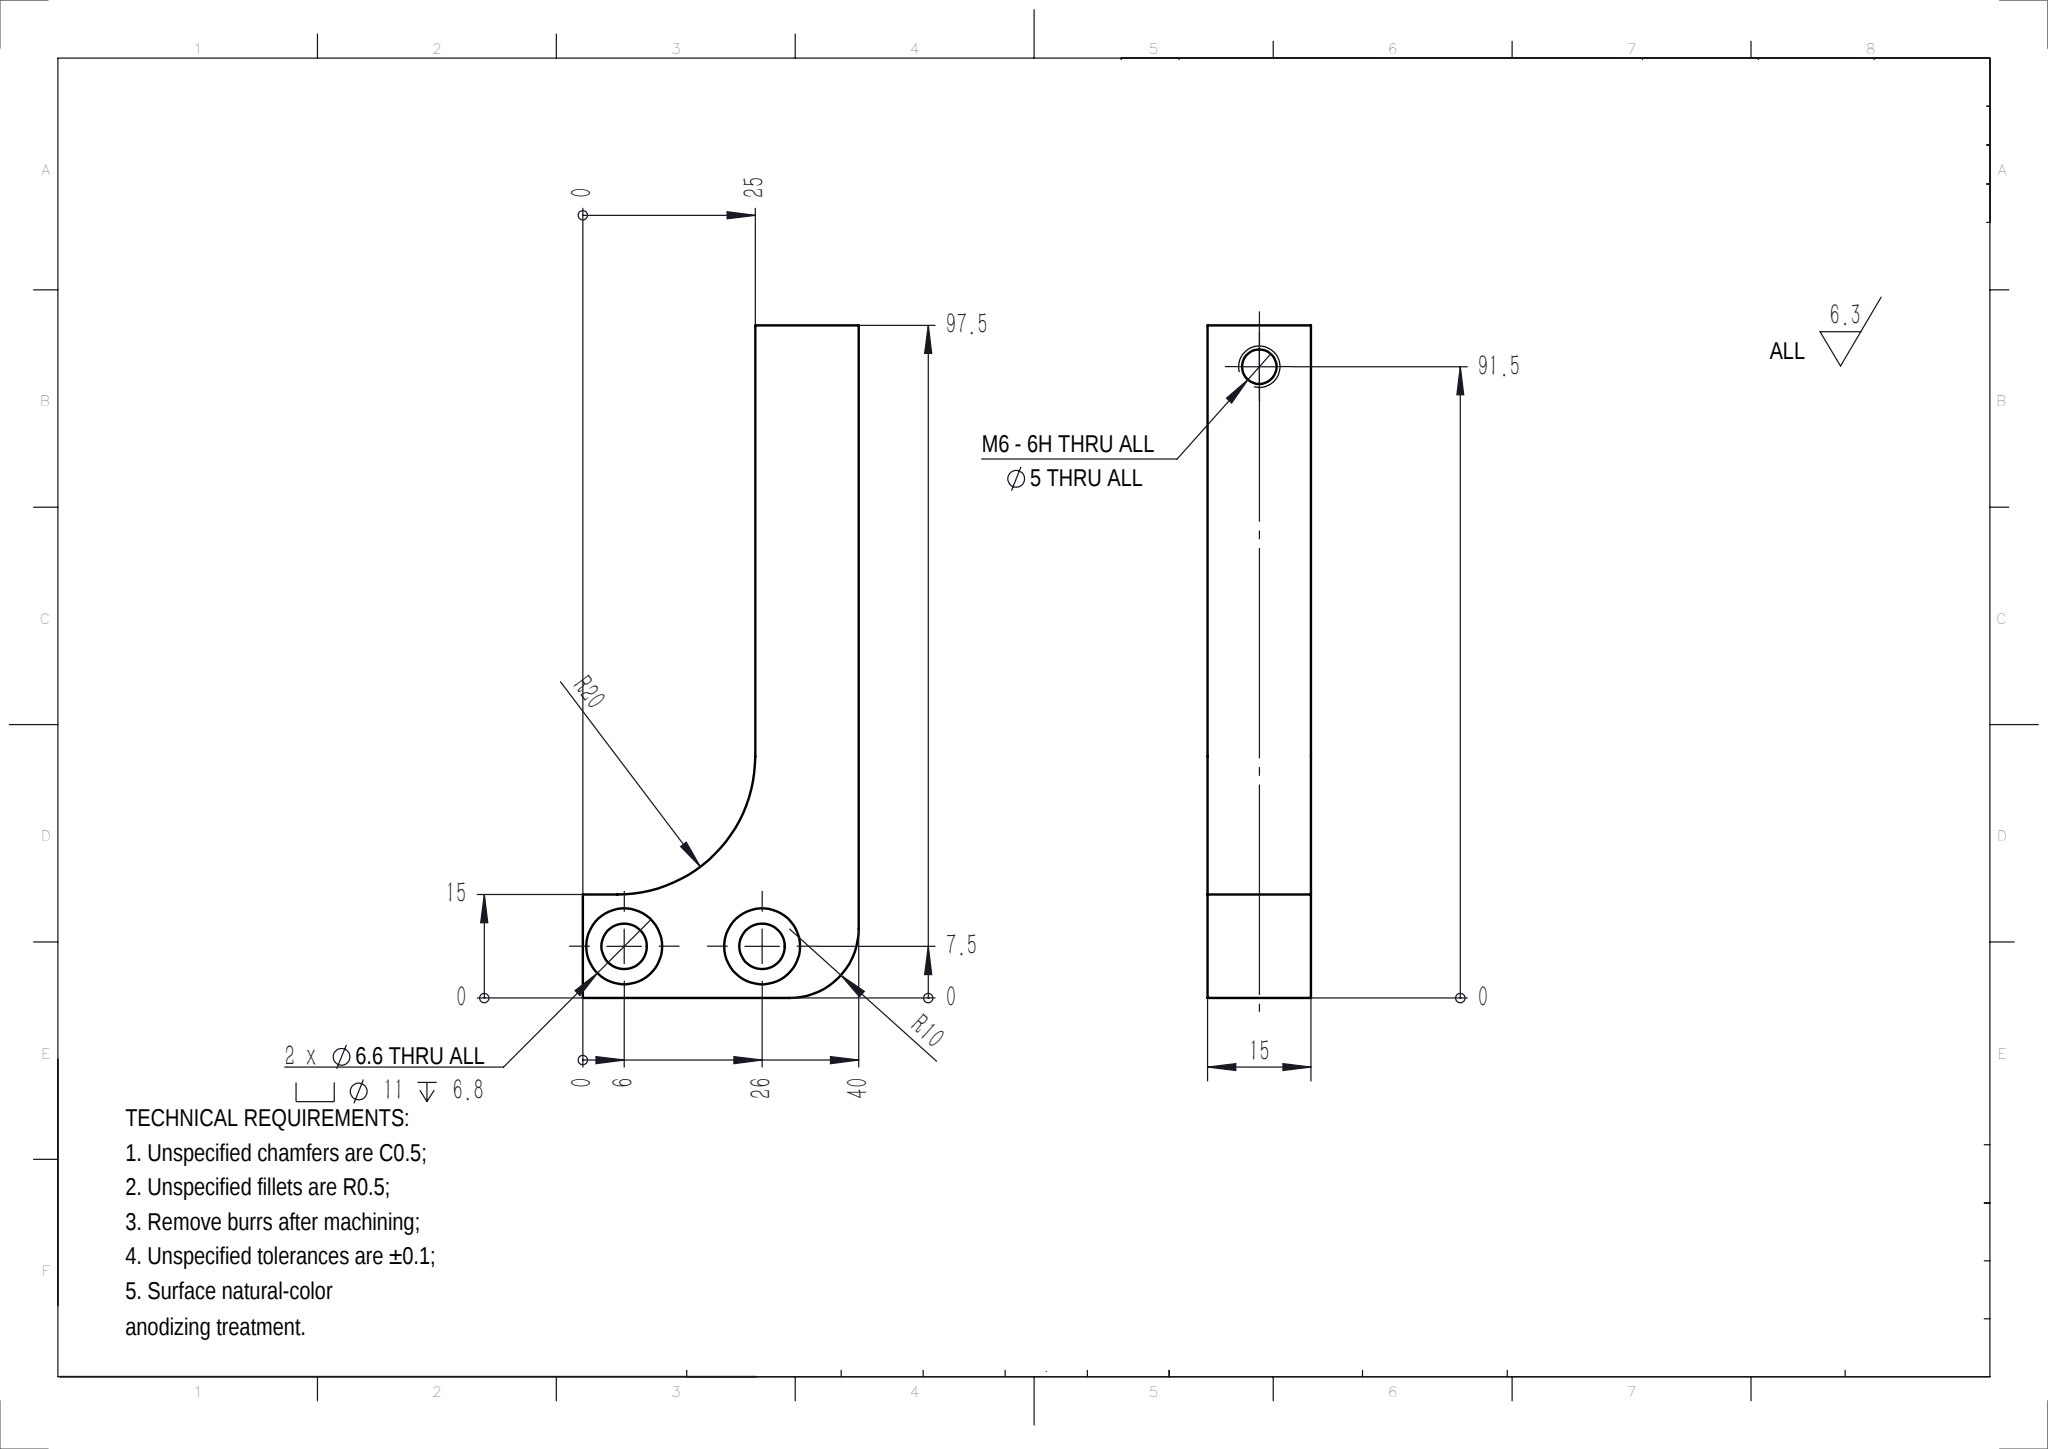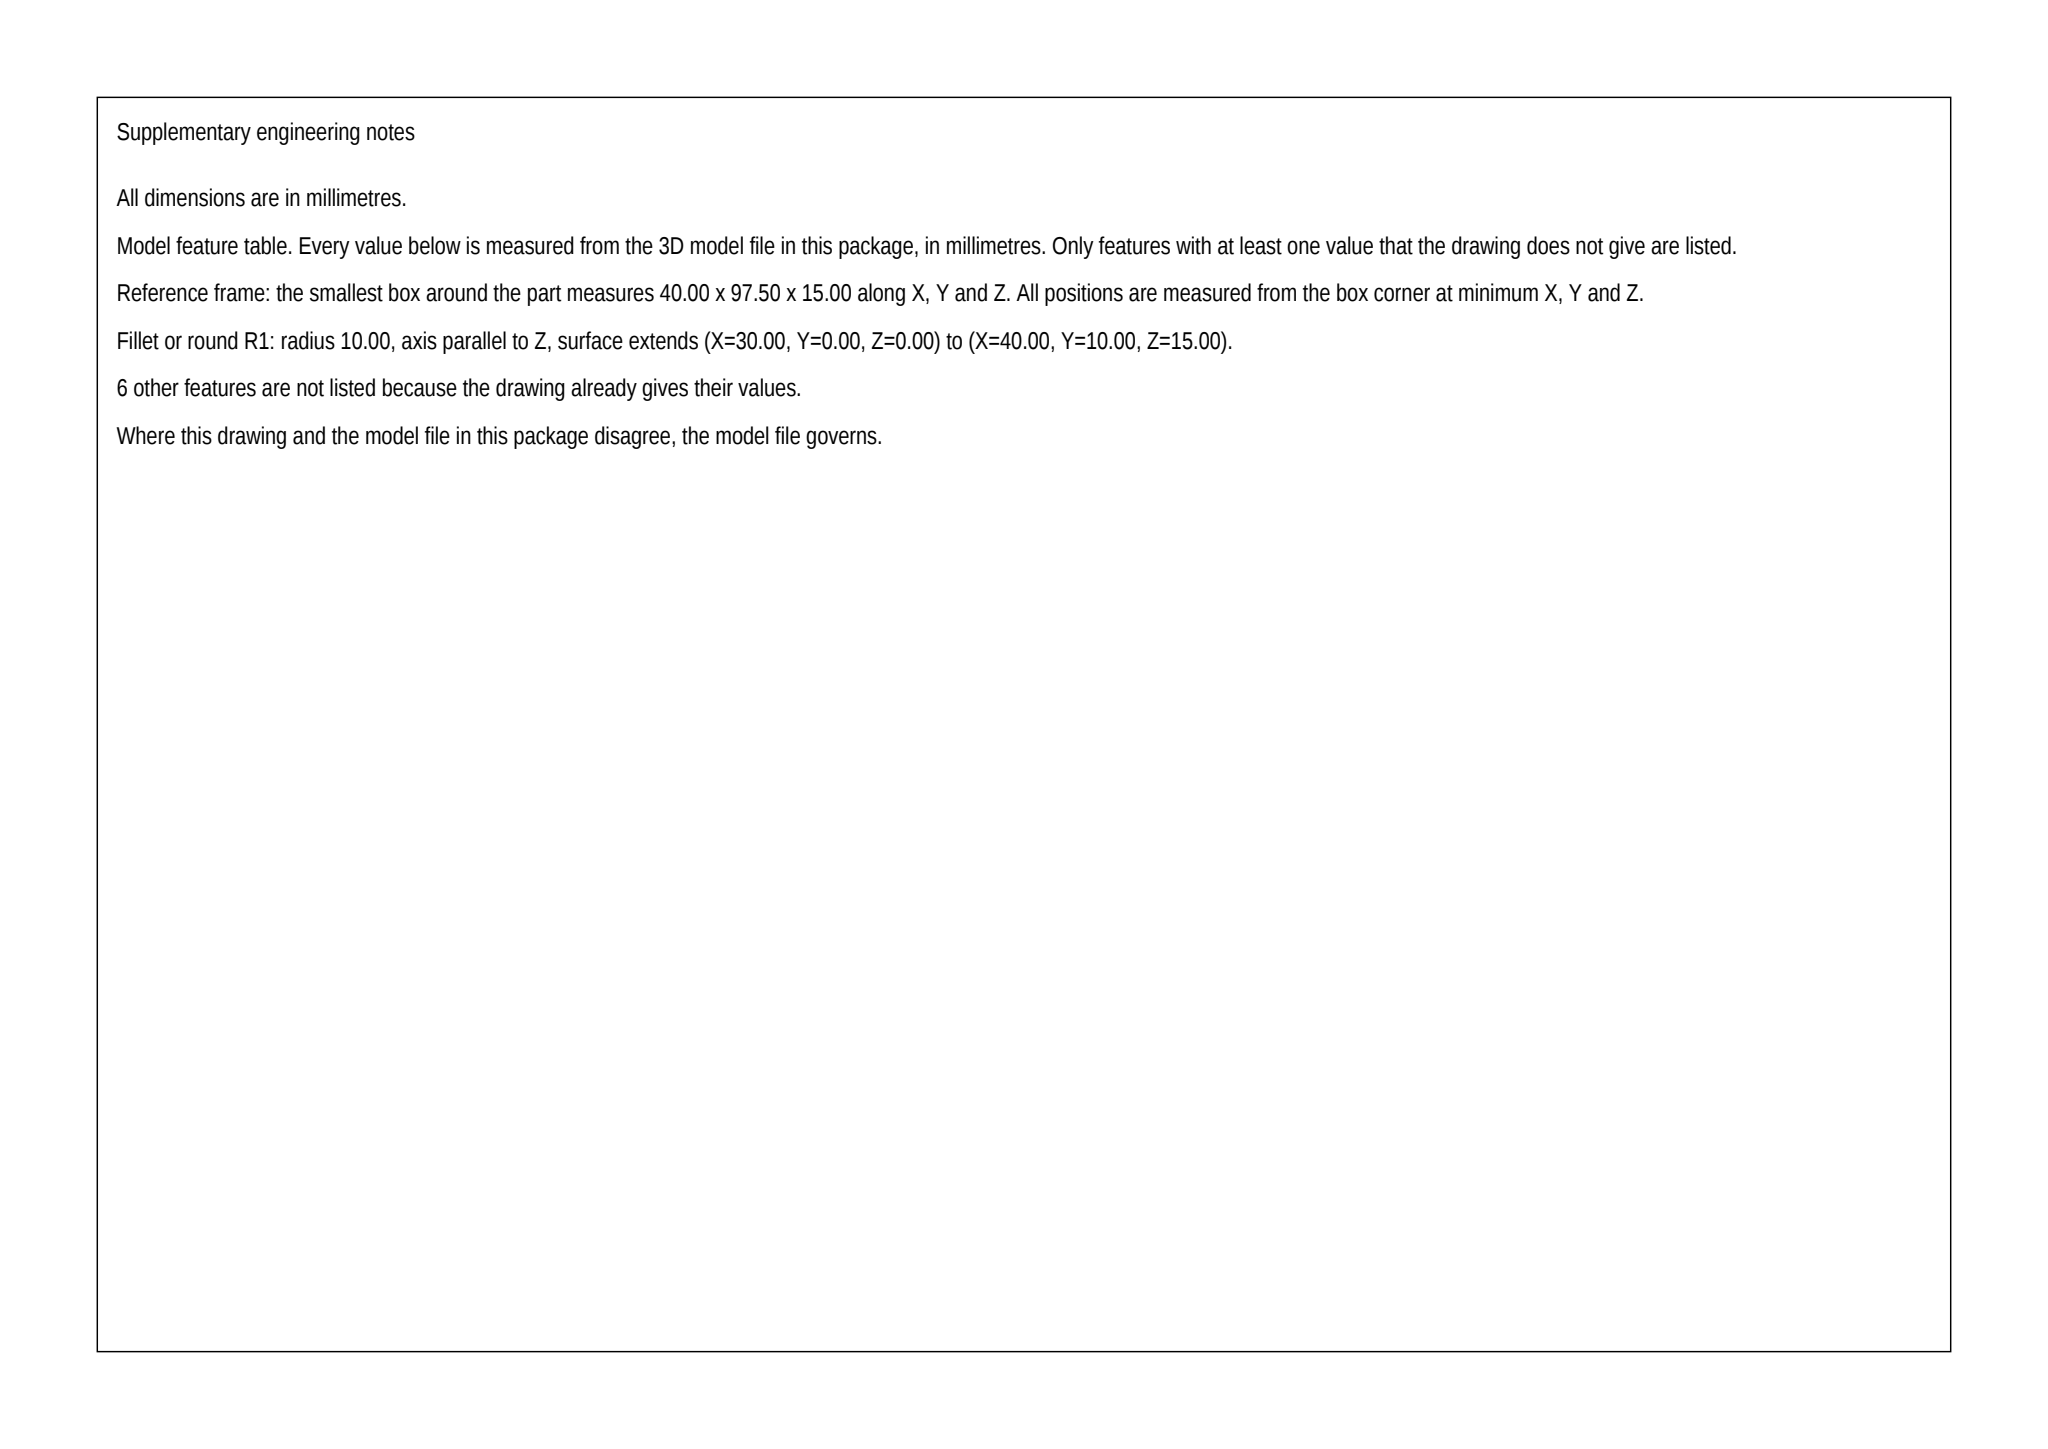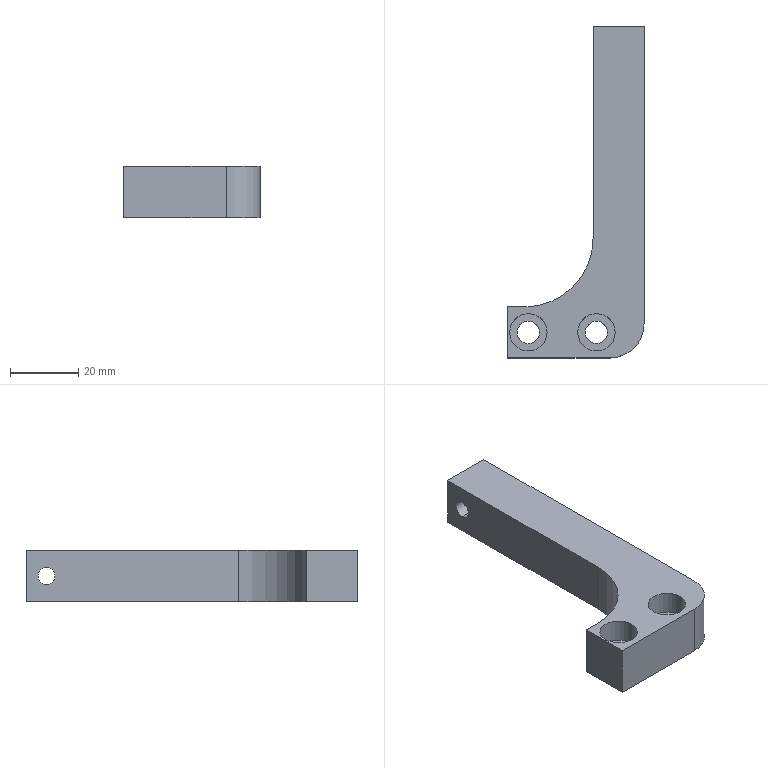Part | SolidWorks | mm | 1 solid | 22 faces | box 40 x 97.5 x 15 mm | volume 26380 mm3 | cylinder 12 | plane 10 | commonest cylinder face diameters 11 x4 6.6 x4 5 x2 40 x1 20 x1
build123d program:
from build123d import *

# Parameters (mm, degrees)
BOSS_EXTRUDE1_DEPTH                               = 7.5
HOLE_SIZE_ACCORDING_TO_HEXAGON_SOCKET_D           = 6.6
HOLE_SIZE_ACCORDING_TO_HEXAGON_SOCKET_CBORE_D     = 11
HOLE_SIZE_ACCORDING_TO_HEXAGON_SOCKET_CBORE_DEPTH = 6.8
M6_TAPPED_HOLE1_D                                 = 5
FILLET1_R                                         = 20
FILLET2_R                                         = 10


with BuildPart() as part:
    # Sketch1 → Boss-Extrude1 (new, symmetric)
    with BuildSketch(Plane.XY):
        Polygon((0, 0), (40, 0), (40, 97.5), (25, 97.5), (25, 15), (0, 15), align=None)
    extrude(amount=BOSS_EXTRUDE1_DEPTH, both=True)

    # Hole Size _ according to_ Hexagon Socket (through all)
    with Locations(Plane.XY.offset(7.5)):
        with Locations((6, 7.5), (26, 7.5)):
            CounterBoreHole(HOLE_SIZE_ACCORDING_TO_HEXAGON_SOCKET_D / 2, HOLE_SIZE_ACCORDING_TO_HEXAGON_SOCKET_CBORE_D / 2, HOLE_SIZE_ACCORDING_TO_HEXAGON_SOCKET_CBORE_DEPTH)

    # M6 Tapped Hole1 (through all)
    with Locations(Plane(origin=(40, 0, 0), x_dir=(0, 0, -1), z_dir=(1, 0, 0))):
        with Locations((0, 91.5)):
            Hole(M6_TAPPED_HOLE1_D / 2)

    # Fillet1
    fillet1_edges = [part.edges().sort_by_distance(p)[0] for p in [
        (25, 15, 0),
    ]]
    fillet(fillet1_edges, radius=FILLET1_R)

    # Fillet2
    fillet2_edges = [part.edges().sort_by_distance(p)[0] for p in [
        (40, 0, 0),
    ]]
    fillet(fillet2_edges, radius=FILLET2_R)


solid = part.part
STEP:
#1=CARTESIAN_POINT('',(25.,91.5,2.5));
#2=VERTEX_POINT('',#1);
#3=CARTESIAN_POINT('',(25.,91.5,-2.5));
#4=VERTEX_POINT('',#3);
#5=CARTESIAN_POINT('',(25.,91.5,0.));
#6=DIRECTION('',(1.,0.,0.));
#7=DIRECTION('',(0.,1.,0.));
#8=AXIS2_PLACEMENT_3D('',#5,#6,#7);
#9=CIRCLE('',#8,2.5);
#10=EDGE_CURVE('',#2,#4,#9,.T.);
#11=ORIENTED_EDGE('',*,*,#10,.F.);
#12=CARTESIAN_POINT('',(40.,91.5,2.5));
#13=VERTEX_POINT('',#12);
#14=CARTESIAN_POINT('',(40.,91.5,2.5));
#15=DIRECTION('',(1.,0.,0.));
#16=VECTOR('',#15,1000.);
#17=LINE('',#14,#16);
#18=EDGE_CURVE('',#2,#13,#17,.T.);
#19=ORIENTED_EDGE('',*,*,#18,.T.);
#20=CARTESIAN_POINT('',(40.,91.5,-2.5));
#21=VERTEX_POINT('',#20);
#22=CARTESIAN_POINT('',(40.,91.5,0.));
#23=DIRECTION('',(1.,0.,0.));
#24=DIRECTION('',(0.,0.,-1.));
#25=AXIS2_PLACEMENT_3D('',#22,#23,#24);
#26=CIRCLE('',#25,2.5);
#27=EDGE_CURVE('',#13,#21,#26,.T.);
#28=ORIENTED_EDGE('',*,*,#27,.T.);
#29=CARTESIAN_POINT('',(40.,91.5,-2.5));
#30=DIRECTION('',(1.,0.,0.));
#31=VECTOR('',#30,1000.);
#32=LINE('',#29,#31);
#33=EDGE_CURVE('',#4,#21,#32,.T.);
#34=ORIENTED_EDGE('',*,*,#33,.F.);
#35=EDGE_LOOP('',(#11,#19,#28,#34));
#36=FACE_OUTER_BOUND('',#35,.T.);
#37=CARTESIAN_POINT('',(40.,91.5,0.));
#38=DIRECTION('',(1.,0.,0.));
#39=DIRECTION('',(0.,0.,-1.));
#40=AXIS2_PLACEMENT_3D('',#37,#38,#39);
#41=CYLINDRICAL_SURFACE('',#40,2.5);
#42=ADVANCED_FACE('',(#36),#41,.F.);
#43=CARTESIAN_POINT('',(0.5,7.5,0.7));
#44=VERTEX_POINT('',#43);
#45=CARTESIAN_POINT('',(11.5,7.5,0.7));
#46=VERTEX_POINT('',#45);
#47=CARTESIAN_POINT('',(6.,7.5,0.7));
#48=DIRECTION('',(0.,0.,1.));
#49=DIRECTION('',(1.,0.,0.));
#50=AXIS2_PLACEMENT_3D('',#47,#48,#49);
#51=CIRCLE('',#50,5.5);
#52=EDGE_CURVE('',#44,#46,#51,.T.);
#53=ORIENTED_EDGE('',*,*,#52,.F.);
#54=CARTESIAN_POINT('',(0.5,7.5,7.5));
#55=VERTEX_POINT('',#54);
#56=CARTESIAN_POINT('',(0.5,7.5,7.5));
#57=DIRECTION('',(0.,0.,1.));
#58=VECTOR('',#57,1000.);
#59=LINE('',#56,#58);
#60=EDGE_CURVE('',#44,#55,#59,.T.);
#61=ORIENTED_EDGE('',*,*,#60,.T.);
#62=CARTESIAN_POINT('',(11.5,7.5,7.5));
#63=VERTEX_POINT('',#62);
#64=CARTESIAN_POINT('',(6.,7.5,7.5));
#65=DIRECTION('',(0.,0.,1.));
#66=DIRECTION('',(1.,0.,0.));
#67=AXIS2_PLACEMENT_3D('',#64,#65,#66);
#68=CIRCLE('',#67,5.5);
#69=EDGE_CURVE('',#55,#63,#68,.T.);
#70=ORIENTED_EDGE('',*,*,#69,.T.);
#71=CARTESIAN_POINT('',(11.5,7.5,7.5));
#72=DIRECTION('',(0.,0.,1.));
#73=VECTOR('',#72,1000.);
#74=LINE('',#71,#73);
#75=EDGE_CURVE('',#46,#63,#74,.T.);
#76=ORIENTED_EDGE('',*,*,#75,.F.);
#77=EDGE_LOOP('',(#53,#61,#70,#76));
#78=FACE_OUTER_BOUND('',#77,.T.);
#79=CARTESIAN_POINT('',(6.,7.5,7.5));
#80=DIRECTION('',(0.,0.,1.));
#81=DIRECTION('',(1.,0.,0.));
#82=AXIS2_PLACEMENT_3D('',#79,#80,#81);
#83=CYLINDRICAL_SURFACE('',#82,5.5);
#84=ADVANCED_FACE('',(#78),#83,.F.);
#85=CARTESIAN_POINT('',(2.7,7.5,-7.5));
#86=VERTEX_POINT('',#85);
#87=CARTESIAN_POINT('',(9.3,7.5,-7.5));
#88=VERTEX_POINT('',#87);
#89=CARTESIAN_POINT('',(6.,7.5,-7.5));
#90=DIRECTION('',(0.,0.,1.));
#91=DIRECTION('',(1.,0.,0.));
#92=AXIS2_PLACEMENT_3D('',#89,#90,#91);
#93=CIRCLE('',#92,3.3);
#94=EDGE_CURVE('',#86,#88,#93,.T.);
#95=ORIENTED_EDGE('',*,*,#94,.F.);
#96=CARTESIAN_POINT('',(2.7,7.5,0.7));
#97=VERTEX_POINT('',#96);
#98=CARTESIAN_POINT('',(2.7,7.5,7.5));
#99=DIRECTION('',(0.,0.,1.));
#100=VECTOR('',#99,1000.);
#101=LINE('',#98,#100);
#102=EDGE_CURVE('',#86,#97,#101,.T.);
#103=ORIENTED_EDGE('',*,*,#102,.T.);
#104=CARTESIAN_POINT('',(9.3,7.5,0.7));
#105=VERTEX_POINT('',#104);
#106=CARTESIAN_POINT('',(6.,7.5,0.7));
#107=DIRECTION('',(0.,0.,1.));
#108=DIRECTION('',(1.,0.,0.));
#109=AXIS2_PLACEMENT_3D('',#106,#107,#108);
#110=CIRCLE('',#109,3.3);
#111=EDGE_CURVE('',#97,#105,#110,.T.);
#112=ORIENTED_EDGE('',*,*,#111,.T.);
#113=CARTESIAN_POINT('',(9.3,7.5,7.5));
#114=DIRECTION('',(0.,0.,1.));
#115=VECTOR('',#114,1000.);
#116=LINE('',#113,#115);
#117=EDGE_CURVE('',#88,#105,#116,.T.);
#118=ORIENTED_EDGE('',*,*,#117,.F.);
#119=EDGE_LOOP('',(#95,#103,#112,#118));
#120=FACE_OUTER_BOUND('',#119,.T.);
#121=CARTESIAN_POINT('',(6.,7.5,7.5));
#122=DIRECTION('',(0.,0.,1.));
#123=DIRECTION('',(1.,0.,0.));
#124=AXIS2_PLACEMENT_3D('',#121,#122,#123);
#125=CYLINDRICAL_SURFACE('',#124,3.3);
#126=ADVANCED_FACE('',(#120),#125,.F.);
#127=CARTESIAN_POINT('',(20.5,7.5,0.7));
#128=VERTEX_POINT('',#127);
#129=CARTESIAN_POINT('',(31.5,7.5,0.7));
#130=VERTEX_POINT('',#129);
#131=CARTESIAN_POINT('',(26.,7.5,0.7));
#132=DIRECTION('',(0.,0.,1.));
#133=DIRECTION('',(1.,0.,0.));
#134=AXIS2_PLACEMENT_3D('',#131,#132,#133);
#135=CIRCLE('',#134,5.5);
#136=EDGE_CURVE('',#128,#130,#135,.T.);
#137=ORIENTED_EDGE('',*,*,#136,.F.);
#138=CARTESIAN_POINT('',(20.5,7.5,7.5));
#139=VERTEX_POINT('',#138);
#140=CARTESIAN_POINT('',(20.5,7.5,7.5));
#141=DIRECTION('',(0.,0.,1.));
#142=VECTOR('',#141,1000.);
#143=LINE('',#140,#142);
#144=EDGE_CURVE('',#128,#139,#143,.T.);
#145=ORIENTED_EDGE('',*,*,#144,.T.);
#146=CARTESIAN_POINT('',(31.5,7.5,7.5));
#147=VERTEX_POINT('',#146);
#148=CARTESIAN_POINT('',(26.,7.5,7.5));
#149=DIRECTION('',(0.,0.,1.));
#150=DIRECTION('',(1.,0.,0.));
#151=AXIS2_PLACEMENT_3D('',#148,#149,#150);
#152=CIRCLE('',#151,5.5);
#153=EDGE_CURVE('',#139,#147,#152,.T.);
#154=ORIENTED_EDGE('',*,*,#153,.T.);
#155=CARTESIAN_POINT('',(31.5,7.5,7.5));
#156=DIRECTION('',(0.,0.,1.));
#157=VECTOR('',#156,1000.);
#158=LINE('',#155,#157);
#159=EDGE_CURVE('',#130,#147,#158,.T.);
#160=ORIENTED_EDGE('',*,*,#159,.F.);
#161=EDGE_LOOP('',(#137,#145,#154,#160));
#162=FACE_OUTER_BOUND('',#161,.T.);
#163=CARTESIAN_POINT('',(26.,7.5,7.5));
#164=DIRECTION('',(0.,0.,1.));
#165=DIRECTION('',(1.,0.,0.));
#166=AXIS2_PLACEMENT_3D('',#163,#164,#165);
#167=CYLINDRICAL_SURFACE('',#166,5.5);
#168=ADVANCED_FACE('',(#162),#167,.F.);
#169=CARTESIAN_POINT('',(22.7,7.5,-7.5));
#170=VERTEX_POINT('',#169);
#171=CARTESIAN_POINT('',(29.3,7.5,-7.5));
#172=VERTEX_POINT('',#171);
#173=CARTESIAN_POINT('',(26.,7.5,-7.5));
#174=DIRECTION('',(0.,0.,1.));
#175=DIRECTION('',(1.,0.,0.));
#176=AXIS2_PLACEMENT_3D('',#173,#174,#175);
#177=CIRCLE('',#176,3.3);
#178=EDGE_CURVE('',#170,#172,#177,.T.);
#179=ORIENTED_EDGE('',*,*,#178,.F.);
#180=CARTESIAN_POINT('',(22.7,7.5,0.7));
#181=VERTEX_POINT('',#180);
#182=CARTESIAN_POINT('',(22.7,7.5,7.5));
#183=DIRECTION('',(0.,0.,1.));
#184=VECTOR('',#183,1000.);
#185=LINE('',#182,#184);
#186=EDGE_CURVE('',#170,#181,#185,.T.);
#187=ORIENTED_EDGE('',*,*,#186,.T.);
#188=CARTESIAN_POINT('',(29.3,7.5,0.7));
#189=VERTEX_POINT('',#188);
#190=CARTESIAN_POINT('',(26.,7.5,0.7));
#191=DIRECTION('',(0.,0.,1.));
#192=DIRECTION('',(1.,0.,0.));
#193=AXIS2_PLACEMENT_3D('',#190,#191,#192);
#194=CIRCLE('',#193,3.3);
#195=EDGE_CURVE('',#181,#189,#194,.T.);
#196=ORIENTED_EDGE('',*,*,#195,.T.);
#197=CARTESIAN_POINT('',(29.3,7.5,7.5));
#198=DIRECTION('',(0.,0.,1.));
#199=VECTOR('',#198,1000.);
#200=LINE('',#197,#199);
#201=EDGE_CURVE('',#172,#189,#200,.T.);
#202=ORIENTED_EDGE('',*,*,#201,.F.);
#203=EDGE_LOOP('',(#179,#187,#196,#202));
#204=FACE_OUTER_BOUND('',#203,.T.);
#205=CARTESIAN_POINT('',(26.,7.5,7.5));
#206=DIRECTION('',(0.,0.,1.));
#207=DIRECTION('',(1.,0.,0.));
#208=AXIS2_PLACEMENT_3D('',#205,#206,#207);
#209=CYLINDRICAL_SURFACE('',#208,3.3);
#210=ADVANCED_FACE('',(#204),#209,.F.);
#211=CARTESIAN_POINT('',(0.,15.,-7.5));
#212=VERTEX_POINT('',#211);
#213=CARTESIAN_POINT('',(0.,0.,-7.5));
#214=VERTEX_POINT('',#213);
#215=CARTESIAN_POINT('',(0.,15.,-7.5));
#216=DIRECTION('',(0.,-1.,0.));
#217=VECTOR('',#216,1000.);
#218=LINE('',#215,#217);
#219=EDGE_CURVE('',#212,#214,#218,.T.);
#220=ORIENTED_EDGE('',*,*,#219,.T.);
#221=CARTESIAN_POINT('',(0.,0.,7.5));
#222=VERTEX_POINT('',#221);
#223=CARTESIAN_POINT('',(0.,0.,7.5));
#224=DIRECTION('',(0.,0.,-1.));
#225=VECTOR('',#224,1000.);
#226=LINE('',#223,#225);
#227=EDGE_CURVE('',#222,#214,#226,.T.);
#228=ORIENTED_EDGE('',*,*,#227,.F.);
#229=CARTESIAN_POINT('',(0.,15.,7.5));
#230=VERTEX_POINT('',#229);
#231=CARTESIAN_POINT('',(0.,15.,7.5));
#232=DIRECTION('',(0.,-1.,0.));
#233=VECTOR('',#232,1000.);
#234=LINE('',#231,#233);
#235=EDGE_CURVE('',#230,#222,#234,.T.);
#236=ORIENTED_EDGE('',*,*,#235,.F.);
#237=CARTESIAN_POINT('',(0.,15.,7.5));
#238=DIRECTION('',(0.,0.,-1.));
#239=VECTOR('',#238,1000.);
#240=LINE('',#237,#239);
#241=EDGE_CURVE('',#230,#212,#240,.T.);
#242=ORIENTED_EDGE('',*,*,#241,.T.);
#243=EDGE_LOOP('',(#220,#228,#236,#242));
#244=FACE_OUTER_BOUND('',#243,.T.);
#245=CARTESIAN_POINT('',(0.,15.,7.5));
#246=DIRECTION('',(1.,0.,0.));
#247=DIRECTION('',(0.,0.,-1.));
#248=AXIS2_PLACEMENT_3D('',#245,#246,#247);
#249=PLANE('',#248);
#250=ADVANCED_FACE('',(#244),#249,.F.);
#251=CARTESIAN_POINT('',(30.,0.,-7.5));
#252=VERTEX_POINT('',#251);
#253=CARTESIAN_POINT('',(0.,0.,-7.5));
#254=DIRECTION('',(1.,0.,0.));
#255=VECTOR('',#254,1000.);
#256=LINE('',#253,#255);
#257=EDGE_CURVE('',#214,#252,#256,.T.);
#258=ORIENTED_EDGE('',*,*,#257,.T.);
#259=CARTESIAN_POINT('',(30.,0.,7.5));
#260=VERTEX_POINT('',#259);
#261=CARTESIAN_POINT('',(30.,0.,7.5));
#262=DIRECTION('',(0.,0.,1.));
#263=VECTOR('',#262,1000.);
#264=LINE('',#261,#263);
#265=EDGE_CURVE('',#252,#260,#264,.T.);
#266=ORIENTED_EDGE('',*,*,#265,.T.);
#267=CARTESIAN_POINT('',(0.,0.,7.5));
#268=DIRECTION('',(1.,0.,0.));
#269=VECTOR('',#268,1000.);
#270=LINE('',#267,#269);
#271=EDGE_CURVE('',#222,#260,#270,.T.);
#272=ORIENTED_EDGE('',*,*,#271,.F.);
#273=ORIENTED_EDGE('',*,*,#227,.T.);
#274=EDGE_LOOP('',(#258,#266,#272,#273));
#275=FACE_OUTER_BOUND('',#274,.T.);
#276=CARTESIAN_POINT('',(0.,0.,7.5));
#277=DIRECTION('',(0.,1.,0.));
#278=DIRECTION('',(0.,0.,1.));
#279=AXIS2_PLACEMENT_3D('',#276,#277,#278);
#280=PLANE('',#279);
#281=ADVANCED_FACE('',(#275),#280,.F.);
#282=CARTESIAN_POINT('',(40.,91.5,0.));
#283=DIRECTION('',(1.,0.,0.));
#284=DIRECTION('',(0.,0.,-1.));
#285=AXIS2_PLACEMENT_3D('',#282,#283,#284);
#286=CIRCLE('',#285,2.5);
#287=EDGE_CURVE('',#21,#13,#286,.T.);
#288=ORIENTED_EDGE('',*,*,#287,.F.);
#289=ORIENTED_EDGE('',*,*,#27,.F.);
#290=EDGE_LOOP('',(#288,#289));
#291=FACE_BOUND('',#290,.T.);
#292=CARTESIAN_POINT('',(40.,10.,7.5));
#293=VERTEX_POINT('',#292);
#294=CARTESIAN_POINT('',(40.,97.5,7.5));
#295=VERTEX_POINT('',#294);
#296=CARTESIAN_POINT('',(40.,0.,7.5));
#297=DIRECTION('',(0.,1.,0.));
#298=VECTOR('',#297,1000.);
#299=LINE('',#296,#298);
#300=EDGE_CURVE('',#293,#295,#299,.T.);
#301=ORIENTED_EDGE('',*,*,#300,.F.);
#302=CARTESIAN_POINT('',(40.,10.,-7.5));
#303=VERTEX_POINT('',#302);
#304=CARTESIAN_POINT('',(40.,10.,7.5));
#305=DIRECTION('',(0.,0.,-1.));
#306=VECTOR('',#305,1000.);
#307=LINE('',#304,#306);
#308=EDGE_CURVE('',#293,#303,#307,.T.);
#309=ORIENTED_EDGE('',*,*,#308,.T.);
#310=CARTESIAN_POINT('',(40.,97.5,-7.5));
#311=VERTEX_POINT('',#310);
#312=CARTESIAN_POINT('',(40.,0.,-7.5));
#313=DIRECTION('',(0.,1.,0.));
#314=VECTOR('',#313,1000.);
#315=LINE('',#312,#314);
#316=EDGE_CURVE('',#303,#311,#315,.T.);
#317=ORIENTED_EDGE('',*,*,#316,.T.);
#318=CARTESIAN_POINT('',(40.,97.5,7.5));
#319=DIRECTION('',(0.,0.,-1.));
#320=VECTOR('',#319,1000.);
#321=LINE('',#318,#320);
#322=EDGE_CURVE('',#295,#311,#321,.T.);
#323=ORIENTED_EDGE('',*,*,#322,.F.);
#324=EDGE_LOOP('',(#301,#309,#317,#323));
#325=FACE_OUTER_BOUND('',#324,.T.);
#326=CARTESIAN_POINT('',(40.,0.,7.5));
#327=DIRECTION('',(-1.,0.,0.));
#328=DIRECTION('',(0.,0.,1.));
#329=AXIS2_PLACEMENT_3D('',#326,#327,#328);
#330=PLANE('',#329);
#331=ADVANCED_FACE('',(#291,#325),#330,.F.);
#332=CARTESIAN_POINT('',(25.,97.5,-7.5));
#333=VERTEX_POINT('',#332);
#334=CARTESIAN_POINT('',(40.,97.5,-7.5));
#335=DIRECTION('',(-1.,0.,0.));
#336=VECTOR('',#335,1000.);
#337=LINE('',#334,#336);
#338=EDGE_CURVE('',#311,#333,#337,.T.);
#339=ORIENTED_EDGE('',*,*,#338,.T.);
#340=CARTESIAN_POINT('',(25.,97.5,7.5));
#341=VERTEX_POINT('',#340);
#342=CARTESIAN_POINT('',(25.,97.5,7.5));
#343=DIRECTION('',(0.,0.,-1.));
#344=VECTOR('',#343,1000.);
#345=LINE('',#342,#344);
#346=EDGE_CURVE('',#341,#333,#345,.T.);
#347=ORIENTED_EDGE('',*,*,#346,.F.);
#348=CARTESIAN_POINT('',(40.,97.5,7.5));
#349=DIRECTION('',(-1.,0.,0.));
#350=VECTOR('',#349,1000.);
#351=LINE('',#348,#350);
#352=EDGE_CURVE('',#295,#341,#351,.T.);
#353=ORIENTED_EDGE('',*,*,#352,.F.);
#354=ORIENTED_EDGE('',*,*,#322,.T.);
#355=EDGE_LOOP('',(#339,#347,#353,#354));
#356=FACE_OUTER_BOUND('',#355,.T.);
#357=CARTESIAN_POINT('',(40.,97.5,7.5));
#358=DIRECTION('',(0.,-1.,0.));
#359=DIRECTION('',(0.,0.,-1.));
#360=AXIS2_PLACEMENT_3D('',#357,#358,#359);
#361=PLANE('',#360);
#362=ADVANCED_FACE('',(#356),#361,.F.);
#363=CARTESIAN_POINT('',(25.,91.5,0.));
#364=DIRECTION('',(1.,0.,0.));
#365=DIRECTION('',(0.,1.,0.));
#366=AXIS2_PLACEMENT_3D('',#363,#364,#365);
#367=CIRCLE('',#366,2.5);
#368=EDGE_CURVE('',#4,#2,#367,.T.);
#369=ORIENTED_EDGE('',*,*,#368,.T.);
#370=ORIENTED_EDGE('',*,*,#10,.T.);
#371=EDGE_LOOP('',(#369,#370));
#372=FACE_BOUND('',#371,.T.);
#373=CARTESIAN_POINT('',(25.,35.,-7.5));
#374=VERTEX_POINT('',#373);
#375=CARTESIAN_POINT('',(25.,97.5,-7.5));
#376=DIRECTION('',(0.,-1.,0.));
#377=VECTOR('',#376,1000.);
#378=LINE('',#375,#377);
#379=EDGE_CURVE('',#333,#374,#378,.T.);
#380=ORIENTED_EDGE('',*,*,#379,.T.);
#381=CARTESIAN_POINT('',(25.,35.,7.5));
#382=VERTEX_POINT('',#381);
#383=CARTESIAN_POINT('',(25.,35.,7.5));
#384=DIRECTION('',(0.,0.,1.));
#385=VECTOR('',#384,1000.);
#386=LINE('',#383,#385);
#387=EDGE_CURVE('',#374,#382,#386,.T.);
#388=ORIENTED_EDGE('',*,*,#387,.T.);
#389=CARTESIAN_POINT('',(25.,97.5,7.5));
#390=DIRECTION('',(0.,-1.,0.));
#391=VECTOR('',#390,1000.);
#392=LINE('',#389,#391);
#393=EDGE_CURVE('',#341,#382,#392,.T.);
#394=ORIENTED_EDGE('',*,*,#393,.F.);
#395=ORIENTED_EDGE('',*,*,#346,.T.);
#396=EDGE_LOOP('',(#380,#388,#394,#395));
#397=FACE_OUTER_BOUND('',#396,.T.);
#398=CARTESIAN_POINT('',(25.,97.5,7.5));
#399=DIRECTION('',(1.,0.,0.));
#400=DIRECTION('',(-0.,1.,0.));
#401=AXIS2_PLACEMENT_3D('',#398,#399,#400);
#402=PLANE('',#401);
#403=ADVANCED_FACE('',(#372,#397),#402,.F.);
#404=CARTESIAN_POINT('',(5.,15.,7.5));
#405=VERTEX_POINT('',#404);
#406=CARTESIAN_POINT('',(25.,15.,7.5));
#407=DIRECTION('',(-1.,-0.,0.));
#408=VECTOR('',#407,1000.);
#409=LINE('',#406,#408);
#410=EDGE_CURVE('',#405,#230,#409,.T.);
#411=ORIENTED_EDGE('',*,*,#410,.F.);
#412=CARTESIAN_POINT('',(5.,15.,-7.5));
#413=VERTEX_POINT('',#412);
#414=CARTESIAN_POINT('',(5.,15.,-7.5));
#415=DIRECTION('',(0.,0.,-1.));
#416=VECTOR('',#415,1000.);
#417=LINE('',#414,#416);
#418=EDGE_CURVE('',#405,#413,#417,.T.);
#419=ORIENTED_EDGE('',*,*,#418,.T.);
#420=CARTESIAN_POINT('',(25.,15.,-7.5));
#421=DIRECTION('',(-1.,-0.,0.));
#422=VECTOR('',#421,1000.);
#423=LINE('',#420,#422);
#424=EDGE_CURVE('',#413,#212,#423,.T.);
#425=ORIENTED_EDGE('',*,*,#424,.T.);
#426=ORIENTED_EDGE('',*,*,#241,.F.);
#427=EDGE_LOOP('',(#411,#419,#425,#426));
#428=FACE_OUTER_BOUND('',#427,.T.);
#429=CARTESIAN_POINT('',(25.,15.,7.5));
#430=DIRECTION('',(0.,-1.,0.));
#431=DIRECTION('',(1.,0.,0.));
#432=AXIS2_PLACEMENT_3D('',#429,#430,#431);
#433=PLANE('',#432);
#434=ADVANCED_FACE('',(#428),#433,.F.);
#435=CARTESIAN_POINT('',(6.,7.5,7.5));
#436=DIRECTION('',(0.,0.,1.));
#437=DIRECTION('',(1.,0.,0.));
#438=AXIS2_PLACEMENT_3D('',#435,#436,#437);
#439=CIRCLE('',#438,5.5);
#440=EDGE_CURVE('',#63,#55,#439,.T.);
#441=ORIENTED_EDGE('',*,*,#440,.F.);
#442=ORIENTED_EDGE('',*,*,#69,.F.);
#443=EDGE_LOOP('',(#441,#442));
#444=FACE_BOUND('',#443,.T.);
#445=CARTESIAN_POINT('',(26.,7.5,7.5));
#446=DIRECTION('',(0.,0.,1.));
#447=DIRECTION('',(1.,0.,0.));
#448=AXIS2_PLACEMENT_3D('',#445,#446,#447);
#449=CIRCLE('',#448,5.5);
#450=EDGE_CURVE('',#147,#139,#449,.T.);
#451=ORIENTED_EDGE('',*,*,#450,.F.);
#452=ORIENTED_EDGE('',*,*,#153,.F.);
#453=EDGE_LOOP('',(#451,#452));
#454=FACE_BOUND('',#453,.T.);
#455=ORIENTED_EDGE('',*,*,#271,.T.);
#456=CARTESIAN_POINT('',(30.,10.,7.5));
#457=DIRECTION('',(0.,0.,1.));
#458=DIRECTION('',(1.,0.,0.));
#459=AXIS2_PLACEMENT_3D('',#456,#457,#458);
#460=CIRCLE('',#459,10.);
#461=EDGE_CURVE('',#260,#293,#460,.T.);
#462=ORIENTED_EDGE('',*,*,#461,.T.);
#463=ORIENTED_EDGE('',*,*,#300,.T.);
#464=ORIENTED_EDGE('',*,*,#352,.T.);
#465=ORIENTED_EDGE('',*,*,#393,.T.);
#466=CARTESIAN_POINT('',(5.,35.,7.5));
#467=DIRECTION('',(0.,0.,-1.));
#468=DIRECTION('',(1.,0.,0.));
#469=AXIS2_PLACEMENT_3D('',#466,#467,#468);
#470=CIRCLE('',#469,20.);
#471=EDGE_CURVE('',#382,#405,#470,.T.);
#472=ORIENTED_EDGE('',*,*,#471,.T.);
#473=ORIENTED_EDGE('',*,*,#410,.T.);
#474=ORIENTED_EDGE('',*,*,#235,.T.);
#475=EDGE_LOOP('',(#455,#462,#463,#464,#465,#472,#473,#474));
#476=FACE_OUTER_BOUND('',#475,.T.);
#477=CARTESIAN_POINT('',(0.,0.,7.5));
#478=DIRECTION('',(0.,0.,1.));
#479=DIRECTION('',(1.,0.,0.));
#480=AXIS2_PLACEMENT_3D('',#477,#478,#479);
#481=PLANE('',#480);
#482=ADVANCED_FACE('',(#444,#454,#476),#481,.T.);
#483=CARTESIAN_POINT('',(6.,7.5,-7.5));
#484=DIRECTION('',(0.,0.,1.));
#485=DIRECTION('',(1.,0.,0.));
#486=AXIS2_PLACEMENT_3D('',#483,#484,#485);
#487=CIRCLE('',#486,3.3);
#488=EDGE_CURVE('',#88,#86,#487,.T.);
#489=ORIENTED_EDGE('',*,*,#488,.T.);
#490=ORIENTED_EDGE('',*,*,#94,.T.);
#491=EDGE_LOOP('',(#489,#490));
#492=FACE_BOUND('',#491,.T.);
#493=CARTESIAN_POINT('',(26.,7.5,-7.5));
#494=DIRECTION('',(0.,0.,1.));
#495=DIRECTION('',(1.,0.,0.));
#496=AXIS2_PLACEMENT_3D('',#493,#494,#495);
#497=CIRCLE('',#496,3.3);
#498=EDGE_CURVE('',#172,#170,#497,.T.);
#499=ORIENTED_EDGE('',*,*,#498,.T.);
#500=ORIENTED_EDGE('',*,*,#178,.T.);
#501=EDGE_LOOP('',(#499,#500));
#502=FACE_BOUND('',#501,.T.);
#503=ORIENTED_EDGE('',*,*,#316,.F.);
#504=CARTESIAN_POINT('',(30.,10.,-7.5));
#505=DIRECTION('',(0.,0.,-1.));
#506=DIRECTION('',(1.,0.,0.));
#507=AXIS2_PLACEMENT_3D('',#504,#505,#506);
#508=CIRCLE('',#507,10.);
#509=EDGE_CURVE('',#303,#252,#508,.T.);
#510=ORIENTED_EDGE('',*,*,#509,.T.);
#511=ORIENTED_EDGE('',*,*,#257,.F.);
#512=ORIENTED_EDGE('',*,*,#219,.F.);
#513=ORIENTED_EDGE('',*,*,#424,.F.);
#514=CARTESIAN_POINT('',(5.,35.,-7.5));
#515=DIRECTION('',(0.,0.,1.));
#516=DIRECTION('',(1.,0.,0.));
#517=AXIS2_PLACEMENT_3D('',#514,#515,#516);
#518=CIRCLE('',#517,20.);
#519=EDGE_CURVE('',#413,#374,#518,.T.);
#520=ORIENTED_EDGE('',*,*,#519,.T.);
#521=ORIENTED_EDGE('',*,*,#379,.F.);
#522=ORIENTED_EDGE('',*,*,#338,.F.);
#523=EDGE_LOOP('',(#503,#510,#511,#512,#513,#520,#521,#522));
#524=FACE_OUTER_BOUND('',#523,.T.);
#525=CARTESIAN_POINT('',(0.,0.,-7.5));
#526=DIRECTION('',(0.,0.,1.));
#527=DIRECTION('',(1.,0.,0.));
#528=AXIS2_PLACEMENT_3D('',#525,#526,#527);
#529=PLANE('',#528);
#530=ADVANCED_FACE('',(#492,#502,#524),#529,.F.);
#531=ORIENTED_EDGE('',*,*,#186,.F.);
#532=ORIENTED_EDGE('',*,*,#498,.F.);
#533=ORIENTED_EDGE('',*,*,#201,.T.);
#534=CARTESIAN_POINT('',(26.,7.5,0.7));
#535=DIRECTION('',(0.,0.,1.));
#536=DIRECTION('',(1.,0.,0.));
#537=AXIS2_PLACEMENT_3D('',#534,#535,#536);
#538=CIRCLE('',#537,3.3);
#539=EDGE_CURVE('',#189,#181,#538,.T.);
#540=ORIENTED_EDGE('',*,*,#539,.T.);
#541=EDGE_LOOP('',(#531,#532,#533,#540));
#542=FACE_OUTER_BOUND('',#541,.T.);
#543=CARTESIAN_POINT('',(26.,7.5,7.5));
#544=DIRECTION('',(0.,0.,1.));
#545=DIRECTION('',(1.,0.,0.));
#546=AXIS2_PLACEMENT_3D('',#543,#544,#545);
#547=CYLINDRICAL_SURFACE('',#546,3.3);
#548=ADVANCED_FACE('',(#542),#547,.F.);
#549=ORIENTED_EDGE('',*,*,#539,.F.);
#550=ORIENTED_EDGE('',*,*,#195,.F.);
#551=EDGE_LOOP('',(#549,#550));
#552=FACE_BOUND('',#551,.T.);
#553=CARTESIAN_POINT('',(26.,7.5,0.7));
#554=DIRECTION('',(0.,0.,1.));
#555=DIRECTION('',(1.,0.,0.));
#556=AXIS2_PLACEMENT_3D('',#553,#554,#555);
#557=CIRCLE('',#556,5.5);
#558=EDGE_CURVE('',#130,#128,#557,.T.);
#559=ORIENTED_EDGE('',*,*,#558,.T.);
#560=ORIENTED_EDGE('',*,*,#136,.T.);
#561=EDGE_LOOP('',(#559,#560));
#562=FACE_OUTER_BOUND('',#561,.T.);
#563=CARTESIAN_POINT('',(29.3,7.5,0.7));
#564=DIRECTION('',(0.,0.,-1.));
#565=DIRECTION('',(-1.,0.,0.));
#566=AXIS2_PLACEMENT_3D('',#563,#564,#565);
#567=PLANE('',#566);
#568=ADVANCED_FACE('',(#552,#562),#567,.F.);
#569=ORIENTED_EDGE('',*,*,#144,.F.);
#570=ORIENTED_EDGE('',*,*,#558,.F.);
#571=ORIENTED_EDGE('',*,*,#159,.T.);
#572=ORIENTED_EDGE('',*,*,#450,.T.);
#573=EDGE_LOOP('',(#569,#570,#571,#572));
#574=FACE_OUTER_BOUND('',#573,.T.);
#575=CARTESIAN_POINT('',(26.,7.5,7.5));
#576=DIRECTION('',(0.,0.,1.));
#577=DIRECTION('',(1.,0.,0.));
#578=AXIS2_PLACEMENT_3D('',#575,#576,#577);
#579=CYLINDRICAL_SURFACE('',#578,5.5);
#580=ADVANCED_FACE('',(#574),#579,.F.);
#581=ORIENTED_EDGE('',*,*,#102,.F.);
#582=ORIENTED_EDGE('',*,*,#488,.F.);
#583=ORIENTED_EDGE('',*,*,#117,.T.);
#584=CARTESIAN_POINT('',(6.,7.5,0.7));
#585=DIRECTION('',(0.,0.,1.));
#586=DIRECTION('',(1.,0.,0.));
#587=AXIS2_PLACEMENT_3D('',#584,#585,#586);
#588=CIRCLE('',#587,3.3);
#589=EDGE_CURVE('',#105,#97,#588,.T.);
#590=ORIENTED_EDGE('',*,*,#589,.T.);
#591=EDGE_LOOP('',(#581,#582,#583,#590));
#592=FACE_OUTER_BOUND('',#591,.T.);
#593=CARTESIAN_POINT('',(6.,7.5,7.5));
#594=DIRECTION('',(0.,0.,1.));
#595=DIRECTION('',(1.,0.,0.));
#596=AXIS2_PLACEMENT_3D('',#593,#594,#595);
#597=CYLINDRICAL_SURFACE('',#596,3.3);
#598=ADVANCED_FACE('',(#592),#597,.F.);
#599=ORIENTED_EDGE('',*,*,#589,.F.);
#600=ORIENTED_EDGE('',*,*,#111,.F.);
#601=EDGE_LOOP('',(#599,#600));
#602=FACE_BOUND('',#601,.T.);
#603=CARTESIAN_POINT('',(6.,7.5,0.7));
#604=DIRECTION('',(0.,0.,1.));
#605=DIRECTION('',(1.,0.,0.));
#606=AXIS2_PLACEMENT_3D('',#603,#604,#605);
#607=CIRCLE('',#606,5.5);
#608=EDGE_CURVE('',#46,#44,#607,.T.);
#609=ORIENTED_EDGE('',*,*,#608,.T.);
#610=ORIENTED_EDGE('',*,*,#52,.T.);
#611=EDGE_LOOP('',(#609,#610));
#612=FACE_OUTER_BOUND('',#611,.T.);
#613=CARTESIAN_POINT('',(9.3,7.5,0.7));
#614=DIRECTION('',(0.,0.,-1.));
#615=DIRECTION('',(-1.,0.,0.));
#616=AXIS2_PLACEMENT_3D('',#613,#614,#615);
#617=PLANE('',#616);
#618=ADVANCED_FACE('',(#602,#612),#617,.F.);
#619=ORIENTED_EDGE('',*,*,#60,.F.);
#620=ORIENTED_EDGE('',*,*,#608,.F.);
#621=ORIENTED_EDGE('',*,*,#75,.T.);
#622=ORIENTED_EDGE('',*,*,#440,.T.);
#623=EDGE_LOOP('',(#619,#620,#621,#622));
#624=FACE_OUTER_BOUND('',#623,.T.);
#625=CARTESIAN_POINT('',(6.,7.5,7.5));
#626=DIRECTION('',(0.,0.,1.));
#627=DIRECTION('',(1.,0.,0.));
#628=AXIS2_PLACEMENT_3D('',#625,#626,#627);
#629=CYLINDRICAL_SURFACE('',#628,5.5);
#630=ADVANCED_FACE('',(#624),#629,.F.);
#631=ORIENTED_EDGE('',*,*,#18,.F.);
#632=ORIENTED_EDGE('',*,*,#368,.F.);
#633=ORIENTED_EDGE('',*,*,#33,.T.);
#634=ORIENTED_EDGE('',*,*,#287,.T.);
#635=EDGE_LOOP('',(#631,#632,#633,#634));
#636=FACE_OUTER_BOUND('',#635,.T.);
#637=CARTESIAN_POINT('',(40.,91.5,0.));
#638=DIRECTION('',(1.,0.,0.));
#639=DIRECTION('',(0.,0.,-1.));
#640=AXIS2_PLACEMENT_3D('',#637,#638,#639);
#641=CYLINDRICAL_SURFACE('',#640,2.5);
#642=ADVANCED_FACE('',(#636),#641,.F.);
#643=ORIENTED_EDGE('',*,*,#471,.F.);
#644=ORIENTED_EDGE('',*,*,#387,.F.);
#645=ORIENTED_EDGE('',*,*,#519,.F.);
#646=ORIENTED_EDGE('',*,*,#418,.F.);
#647=EDGE_LOOP('',(#643,#644,#645,#646));
#648=FACE_OUTER_BOUND('',#647,.T.);
#649=CARTESIAN_POINT('',(5.,35.,7.5));
#650=DIRECTION('',(0.,0.,1.));
#651=DIRECTION('',(1.,0.,0.));
#652=AXIS2_PLACEMENT_3D('',#649,#650,#651);
#653=CYLINDRICAL_SURFACE('',#652,20.);
#654=ADVANCED_FACE('',(#648),#653,.F.);
#655=ORIENTED_EDGE('',*,*,#461,.F.);
#656=ORIENTED_EDGE('',*,*,#265,.F.);
#657=ORIENTED_EDGE('',*,*,#509,.F.);
#658=ORIENTED_EDGE('',*,*,#308,.F.);
#659=EDGE_LOOP('',(#655,#656,#657,#658));
#660=FACE_OUTER_BOUND('',#659,.T.);
#661=CARTESIAN_POINT('',(30.,10.,7.5));
#662=DIRECTION('',(0.,0.,-1.));
#663=DIRECTION('',(-1.,0.,0.));
#664=AXIS2_PLACEMENT_3D('',#661,#662,#663);
#665=CYLINDRICAL_SURFACE('',#664,10.);
#666=ADVANCED_FACE('',(#660),#665,.T.);
#667=CLOSED_SHELL('',(#42,#84,#126,#168,#210,#250,#281,#331,#362,#403,#434,#482,#530,#548,#568,#580,#598,#618,#630,#642,#654,#666));
#668=MANIFOLD_SOLID_BREP('',#667);
#669=CARTESIAN_POINT('',(0.,0.,0.));
#670=DIRECTION('',(0.,0.,1.));
#671=DIRECTION('',(1.,0.,0.));
#672=AXIS2_PLACEMENT_3D('',#669,#670,#671);
#673=(LENGTH_UNIT()NAMED_UNIT(*)SI_UNIT(.MILLI.,.METRE.));
#674=UNCERTAINTY_MEASURE_WITH_UNIT(LENGTH_MEASURE(0.00001),#673,'','');
#675=(NAMED_UNIT(*)PLANE_ANGLE_UNIT()SI_UNIT($,.RADIAN.));
#676=(NAMED_UNIT(*)SI_UNIT($,.STERADIAN.)SOLID_ANGLE_UNIT());
#677=(GEOMETRIC_REPRESENTATION_CONTEXT(3)GLOBAL_UNCERTAINTY_ASSIGNED_CONTEXT((#674))GLOBAL_UNIT_ASSIGNED_CONTEXT((#673,#675,#676))REPRESENTATION_CONTEXT('',''));
#678=ADVANCED_BREP_SHAPE_REPRESENTATION('',(#668,#672),#677);